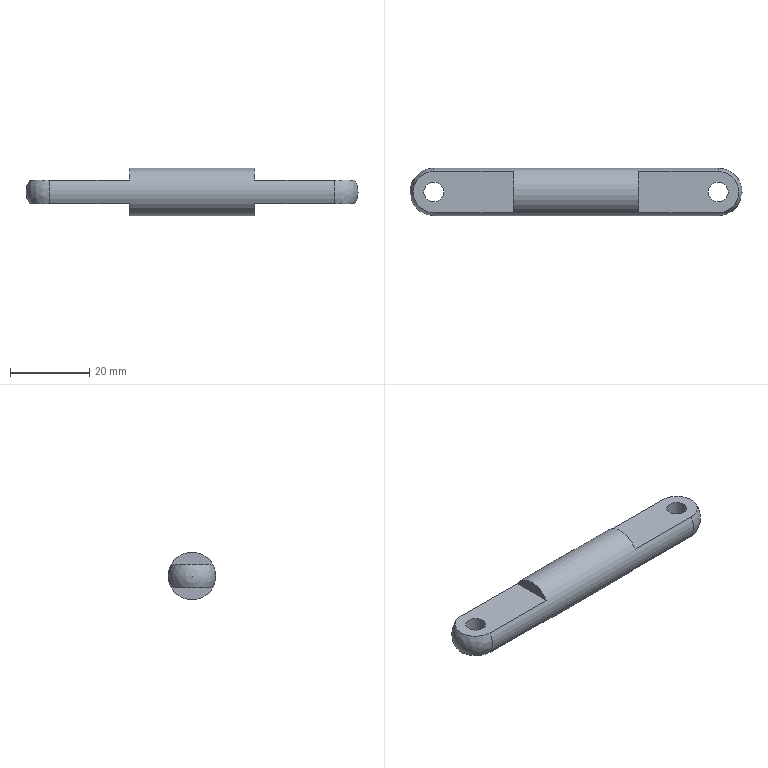Component | NX | HINGE_ROD | 1 solid | 13 faces | volume 6727 mm3 | plane 8 | cylinder 3 | sphere 2 | commonest cylinder face diameters 5 x2 12 x1